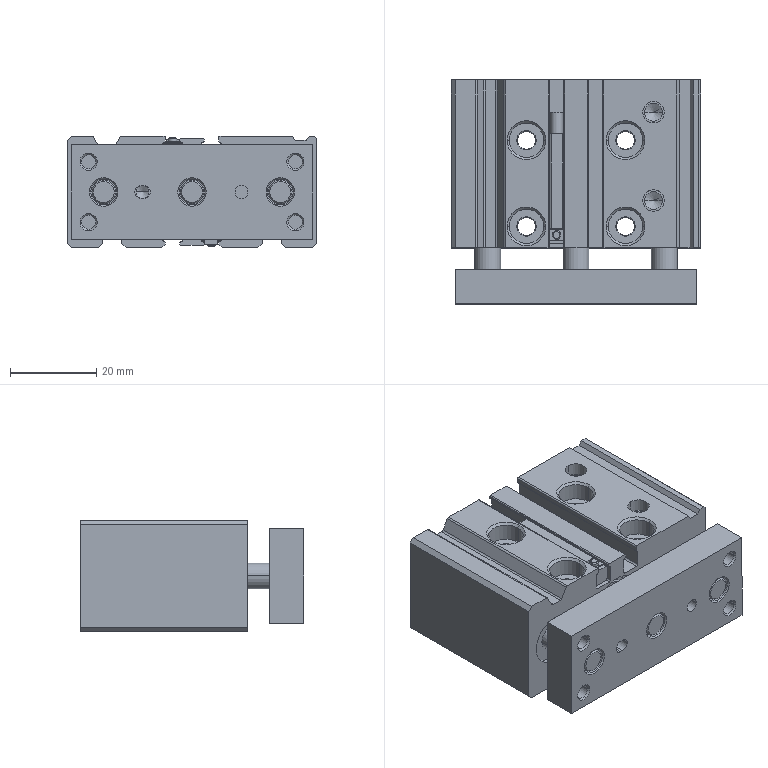Component | SolidWorks | PurchasedPart_Three-axisCylinderTCL12x10S-1 | 4 solids | 437 faces | box 58 x 52 x 26 mm | volume 55062 mm3 | cylinder 193 | plane 156 | cone 86 | torus 2 | commonest cylinder face diameters 3 x25 0.8 x24 6 x18 0.4 x16 3.242 x16 4.134 x12 0.6 x10 12 x10